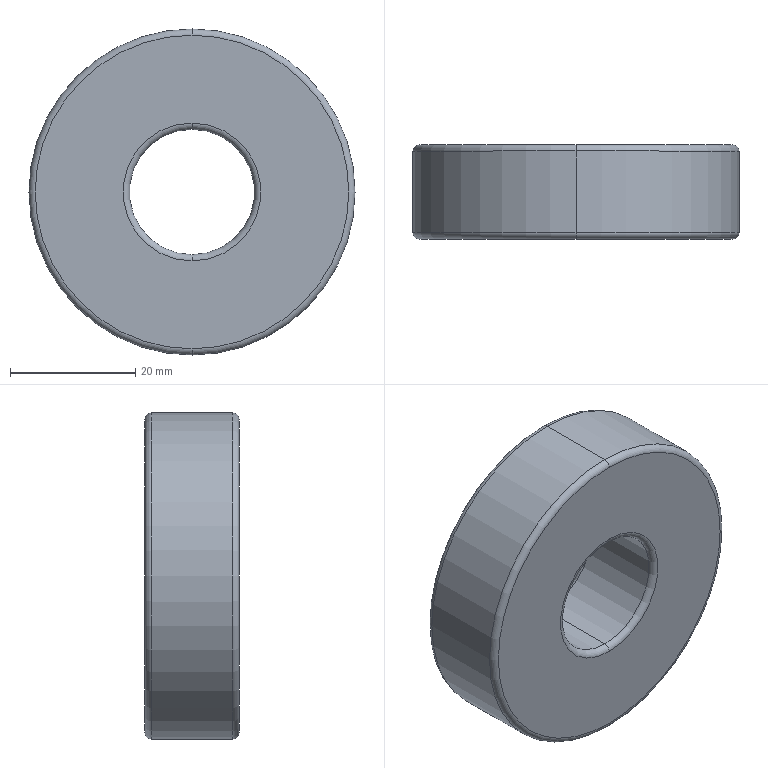Component | SolidWorks | BearingCH-NTN6304ZZ-1 | 1 solid | 14 faces | box 52 x 15 x 52 mm | volume 27046 mm3 | torus 8 | cylinder 4 | plane 2 | commonest cylinder face diameters 20 x2 52 x2
build123d program:
from build123d import *

# Parameters (mm, degrees)
SKETCH1_R           = 26
SKETCH1_R_2         = 10
BOSS_EXTRUDE1_DEPTH = 15
FILLET1_R           = 1


with BuildPart() as part:
    # Sketch1 → Boss-Extrude1 (new body)
    with BuildSketch(Plane(origin=(0, 0, 0), x_dir=(1, 0, 0), z_dir=(0, 1, 0))):
        with Locations(Location((0, 0, 0), (0, 0, 270))):
            Circle(SKETCH1_R)
        with Locations(Location((0, 0, 0), (0, 0, 270))):
            Circle(SKETCH1_R_2, mode=Mode.SUBTRACT)
    extrude(amount=BOSS_EXTRUDE1_DEPTH)

    # Fillet1
    fillet1_edges = [part.edges().sort_by_distance(p)[0] for p in [
        (0, 0, -26),
        (0, 15, -26),
        (0, 0, -10),
        (0, 15, -10),
    ]]
    fillet(fillet1_edges, radius=FILLET1_R)


solid = part.part

# Placed as in the assembly
solid = solid.moved(Location((-30.964, 101.813, 280.197), (0, 0, 0)))
STEP:
#1=COLOUR_RGB('',0.7922,0.8196,0.9333);
#2=FILL_AREA_STYLE_COLOUR('',#1);
#3=FILL_AREA_STYLE('',(#2));
#4=SURFACE_STYLE_FILL_AREA(#3);
#5=SURFACE_SIDE_STYLE('',(#4));
#6=SURFACE_STYLE_USAGE(.BOTH.,#5);
#7=PRESENTATION_STYLE_ASSIGNMENT((#6));
#8=CARTESIAN_POINT('',(-1.219,4.599,10.598));
#9=VERTEX_POINT('',#8);
#10=CARTESIAN_POINT('',(-1.219,4.599,11.464));
#11=VERTEX_POINT('',#10);
#12=CARTESIAN_POINT('',(-1.219,4.599,11.031));
#13=DIRECTION('',(0.,-1.,0.));
#14=DIRECTION('',(0.,0.,1.));
#15=AXIS2_PLACEMENT_3D('',#12,#13,#14);
#16=CIRCLE('',#15,0.4331);
#17=EDGE_CURVE('',#9,#11,#16,.T.);
#18=ORIENTED_EDGE('',*,*,#17,.F.);
#19=CARTESIAN_POINT('',(-1.219,4.56,10.638));
#20=VERTEX_POINT('',#19);
#21=CARTESIAN_POINT('',(-1.219,4.56,10.598));
#22=DIRECTION('',(1.,0.,0.));
#23=DIRECTION('',(0.,0.,-1.));
#24=AXIS2_PLACEMENT_3D('',#21,#22,#23);
#25=CIRCLE('',#24,0.03937);
#26=EDGE_CURVE('',#9,#20,#25,.T.);
#27=ORIENTED_EDGE('',*,*,#26,.T.);
#28=CARTESIAN_POINT('',(-1.219,4.56,11.425));
#29=VERTEX_POINT('',#28);
#30=CARTESIAN_POINT('',(-1.219,4.56,11.031));
#31=DIRECTION('',(0.,1.,0.));
#32=DIRECTION('',(0.,0.,1.));
#33=AXIS2_PLACEMENT_3D('',#30,#31,#32);
#34=CIRCLE('',#33,0.3937);
#35=EDGE_CURVE('',#29,#20,#34,.T.);
#36=ORIENTED_EDGE('',*,*,#35,.F.);
#37=CARTESIAN_POINT('',(-1.219,4.56,11.464));
#38=DIRECTION('',(-1.,0.,0.));
#39=DIRECTION('',(0.,0.,1.));
#40=AXIS2_PLACEMENT_3D('',#37,#38,#39);
#41=CIRCLE('',#40,0.03937);
#42=EDGE_CURVE('',#11,#29,#41,.T.);
#43=ORIENTED_EDGE('',*,*,#42,.F.);
#44=EDGE_LOOP('',(#18,#27,#36,#43));
#45=FACE_OUTER_BOUND('',#44,.T.);
#46=CARTESIAN_POINT('',(-1.219,4.56,11.031));
#47=DIRECTION('',(0.,1.,0.));
#48=DIRECTION('',(0.,0.,1.));
#49=AXIS2_PLACEMENT_3D('',#46,#47,#48);
#50=TOROIDAL_SURFACE('',#49,0.4331,0.03937);
#51=ADVANCED_FACE('',(#45),#50,.T.);
#52=CARTESIAN_POINT('',(-1.219,4.048,10.638));
#53=VERTEX_POINT('',#52);
#54=CARTESIAN_POINT('',(-1.219,4.048,11.425));
#55=VERTEX_POINT('',#54);
#56=CARTESIAN_POINT('',(-1.219,4.048,11.031));
#57=DIRECTION('',(0.,-1.,0.));
#58=DIRECTION('',(0.,0.,1.));
#59=AXIS2_PLACEMENT_3D('',#56,#57,#58);
#60=CIRCLE('',#59,0.3937);
#61=EDGE_CURVE('',#53,#55,#60,.T.);
#62=ORIENTED_EDGE('',*,*,#61,.F.);
#63=CARTESIAN_POINT('',(-1.219,4.008,10.598));
#64=VERTEX_POINT('',#63);
#65=CARTESIAN_POINT('',(-1.219,4.048,10.598));
#66=DIRECTION('',(1.,0.,0.));
#67=DIRECTION('',(0.,0.,-1.));
#68=AXIS2_PLACEMENT_3D('',#65,#66,#67);
#69=CIRCLE('',#68,0.03937);
#70=EDGE_CURVE('',#53,#64,#69,.T.);
#71=ORIENTED_EDGE('',*,*,#70,.T.);
#72=CARTESIAN_POINT('',(-1.219,4.008,11.464));
#73=VERTEX_POINT('',#72);
#74=CARTESIAN_POINT('',(-1.219,4.008,11.031));
#75=DIRECTION('',(0.,1.,0.));
#76=DIRECTION('',(0.,0.,1.));
#77=AXIS2_PLACEMENT_3D('',#74,#75,#76);
#78=CIRCLE('',#77,0.4331);
#79=EDGE_CURVE('',#73,#64,#78,.T.);
#80=ORIENTED_EDGE('',*,*,#79,.F.);
#81=CARTESIAN_POINT('',(-1.219,4.048,11.464));
#82=DIRECTION('',(-1.,0.,0.));
#83=DIRECTION('',(0.,0.,1.));
#84=AXIS2_PLACEMENT_3D('',#81,#82,#83);
#85=CIRCLE('',#84,0.03937);
#86=EDGE_CURVE('',#55,#73,#85,.T.);
#87=ORIENTED_EDGE('',*,*,#86,.F.);
#88=EDGE_LOOP('',(#62,#71,#80,#87));
#89=FACE_OUTER_BOUND('',#88,.T.);
#90=CARTESIAN_POINT('',(-1.219,4.048,11.031));
#91=DIRECTION('',(0.,1.,0.));
#92=DIRECTION('',(0.,0.,1.));
#93=AXIS2_PLACEMENT_3D('',#90,#91,#92);
#94=TOROIDAL_SURFACE('',#93,0.4331,0.03937);
#95=ADVANCED_FACE('',(#89),#94,.T.);
#96=CARTESIAN_POINT('',(-1.219,4.56,10.008));
#97=VERTEX_POINT('',#96);
#98=CARTESIAN_POINT('',(-1.219,4.56,12.055));
#99=VERTEX_POINT('',#98);
#100=CARTESIAN_POINT('',(-1.219,4.56,11.031));
#101=DIRECTION('',(0.,-1.,0.));
#102=DIRECTION('',(0.,0.,1.));
#103=AXIS2_PLACEMENT_3D('',#100,#101,#102);
#104=CIRCLE('',#103,1.024);
#105=EDGE_CURVE('',#97,#99,#104,.T.);
#106=ORIENTED_EDGE('',*,*,#105,.F.);
#107=CARTESIAN_POINT('',(-1.219,4.599,10.047));
#108=VERTEX_POINT('',#107);
#109=CARTESIAN_POINT('',(-1.219,4.56,10.047));
#110=DIRECTION('',(1.,0.,0.));
#111=DIRECTION('',(0.,0.,-1.));
#112=AXIS2_PLACEMENT_3D('',#109,#110,#111);
#113=CIRCLE('',#112,0.03937);
#114=EDGE_CURVE('',#97,#108,#113,.T.);
#115=ORIENTED_EDGE('',*,*,#114,.T.);
#116=CARTESIAN_POINT('',(-1.219,4.599,12.016));
#117=VERTEX_POINT('',#116);
#118=CARTESIAN_POINT('',(-1.219,4.599,11.031));
#119=DIRECTION('',(0.,1.,0.));
#120=DIRECTION('',(0.,0.,1.));
#121=AXIS2_PLACEMENT_3D('',#118,#119,#120);
#122=CIRCLE('',#121,0.9843);
#123=EDGE_CURVE('',#117,#108,#122,.T.);
#124=ORIENTED_EDGE('',*,*,#123,.F.);
#125=CARTESIAN_POINT('',(-1.219,4.56,12.016));
#126=DIRECTION('',(-1.,0.,0.));
#127=DIRECTION('',(0.,0.,1.));
#128=AXIS2_PLACEMENT_3D('',#125,#126,#127);
#129=CIRCLE('',#128,0.03937);
#130=EDGE_CURVE('',#99,#117,#129,.T.);
#131=ORIENTED_EDGE('',*,*,#130,.F.);
#132=EDGE_LOOP('',(#106,#115,#124,#131));
#133=FACE_OUTER_BOUND('',#132,.T.);
#134=CARTESIAN_POINT('',(-1.219,4.56,11.031));
#135=DIRECTION('',(0.,1.,0.));
#136=DIRECTION('',(0.,0.,1.));
#137=AXIS2_PLACEMENT_3D('',#134,#135,#136);
#138=TOROIDAL_SURFACE('',#137,0.9843,0.03937);
#139=ADVANCED_FACE('',(#133),#138,.T.);
#140=CARTESIAN_POINT('',(-1.219,4.008,10.047));
#141=VERTEX_POINT('',#140);
#142=CARTESIAN_POINT('',(-1.219,4.008,12.016));
#143=VERTEX_POINT('',#142);
#144=CARTESIAN_POINT('',(-1.219,4.008,11.031));
#145=DIRECTION('',(0.,-1.,0.));
#146=DIRECTION('',(0.,0.,1.));
#147=AXIS2_PLACEMENT_3D('',#144,#145,#146);
#148=CIRCLE('',#147,0.9843);
#149=EDGE_CURVE('',#141,#143,#148,.T.);
#150=ORIENTED_EDGE('',*,*,#149,.F.);
#151=CARTESIAN_POINT('',(-1.219,4.048,10.008));
#152=VERTEX_POINT('',#151);
#153=CARTESIAN_POINT('',(-1.219,4.048,10.047));
#154=DIRECTION('',(1.,0.,0.));
#155=DIRECTION('',(0.,0.,-1.));
#156=AXIS2_PLACEMENT_3D('',#153,#154,#155);
#157=CIRCLE('',#156,0.03937);
#158=EDGE_CURVE('',#141,#152,#157,.T.);
#159=ORIENTED_EDGE('',*,*,#158,.T.);
#160=CARTESIAN_POINT('',(-1.219,4.048,12.055));
#161=VERTEX_POINT('',#160);
#162=CARTESIAN_POINT('',(-1.219,4.048,11.031));
#163=DIRECTION('',(0.,1.,0.));
#164=DIRECTION('',(0.,0.,1.));
#165=AXIS2_PLACEMENT_3D('',#162,#163,#164);
#166=CIRCLE('',#165,1.024);
#167=EDGE_CURVE('',#161,#152,#166,.T.);
#168=ORIENTED_EDGE('',*,*,#167,.F.);
#169=CARTESIAN_POINT('',(-1.219,4.048,12.016));
#170=DIRECTION('',(-1.,0.,0.));
#171=DIRECTION('',(0.,0.,1.));
#172=AXIS2_PLACEMENT_3D('',#169,#170,#171);
#173=CIRCLE('',#172,0.03937);
#174=EDGE_CURVE('',#143,#161,#173,.T.);
#175=ORIENTED_EDGE('',*,*,#174,.F.);
#176=EDGE_LOOP('',(#150,#159,#168,#175));
#177=FACE_OUTER_BOUND('',#176,.T.);
#178=CARTESIAN_POINT('',(-1.219,4.048,11.031));
#179=DIRECTION('',(0.,1.,0.));
#180=DIRECTION('',(0.,0.,1.));
#181=AXIS2_PLACEMENT_3D('',#178,#179,#180);
#182=TOROIDAL_SURFACE('',#181,0.9843,0.03937);
#183=ADVANCED_FACE('',(#177),#182,.T.);
#184=CARTESIAN_POINT('',(-1.219,4.56,11.031));
#185=DIRECTION('',(0.,1.,0.));
#186=DIRECTION('',(0.,0.,1.));
#187=AXIS2_PLACEMENT_3D('',#184,#185,#186);
#188=CIRCLE('',#187,0.3937);
#189=EDGE_CURVE('',#20,#29,#188,.T.);
#190=ORIENTED_EDGE('',*,*,#189,.T.);
#191=CARTESIAN_POINT('',(-1.219,4.599,11.425));
#192=DIRECTION('',(0.,-1.,0.));
#193=VECTOR('',#192,39.37);
#194=LINE('',#191,#193);
#195=EDGE_CURVE('',#29,#55,#194,.T.);
#196=ORIENTED_EDGE('',*,*,#195,.T.);
#197=CARTESIAN_POINT('',(-1.219,4.048,11.031));
#198=DIRECTION('',(0.,-1.,0.));
#199=DIRECTION('',(0.,0.,1.));
#200=AXIS2_PLACEMENT_3D('',#197,#198,#199);
#201=CIRCLE('',#200,0.3937);
#202=EDGE_CURVE('',#55,#53,#201,.T.);
#203=ORIENTED_EDGE('',*,*,#202,.T.);
#204=CARTESIAN_POINT('',(-1.219,4.599,10.638));
#205=DIRECTION('',(0.,-1.,0.));
#206=VECTOR('',#205,39.37);
#207=LINE('',#204,#206);
#208=EDGE_CURVE('',#20,#53,#207,.T.);
#209=ORIENTED_EDGE('',*,*,#208,.F.);
#210=EDGE_LOOP('',(#190,#196,#203,#209));
#211=FACE_OUTER_BOUND('',#210,.T.);
#212=CARTESIAN_POINT('',(-1.219,4.599,11.031));
#213=DIRECTION('',(0.,-1.,0.));
#214=DIRECTION('',(0.,0.,-1.));
#215=AXIS2_PLACEMENT_3D('',#212,#213,#214);
#216=CYLINDRICAL_SURFACE('',#215,0.3937);
#217=ADVANCED_FACE('',(#211),#216,.F.);
#218=ORIENTED_EDGE('',*,*,#105,.T.);
#219=CARTESIAN_POINT('',(-1.219,4.599,12.055));
#220=DIRECTION('',(0.,-1.,0.));
#221=VECTOR('',#220,39.37);
#222=LINE('',#219,#221);
#223=EDGE_CURVE('',#99,#161,#222,.T.);
#224=ORIENTED_EDGE('',*,*,#223,.T.);
#225=ORIENTED_EDGE('',*,*,#167,.T.);
#226=CARTESIAN_POINT('',(-1.219,4.599,10.008));
#227=DIRECTION('',(0.,-1.,0.));
#228=VECTOR('',#227,39.37);
#229=LINE('',#226,#228);
#230=EDGE_CURVE('',#97,#152,#229,.T.);
#231=ORIENTED_EDGE('',*,*,#230,.F.);
#232=EDGE_LOOP('',(#218,#224,#225,#231));
#233=FACE_OUTER_BOUND('',#232,.T.);
#234=CARTESIAN_POINT('',(-1.219,4.599,11.031));
#235=DIRECTION('',(0.,-1.,0.));
#236=DIRECTION('',(0.,0.,-1.));
#237=AXIS2_PLACEMENT_3D('',#234,#235,#236);
#238=CYLINDRICAL_SURFACE('',#237,1.024);
#239=ADVANCED_FACE('',(#233),#238,.T.);
#240=ORIENTED_EDGE('',*,*,#123,.T.);
#241=CARTESIAN_POINT('',(-1.219,4.599,11.031));
#242=DIRECTION('',(0.,1.,0.));
#243=DIRECTION('',(0.,0.,1.));
#244=AXIS2_PLACEMENT_3D('',#241,#242,#243);
#245=CIRCLE('',#244,0.9843);
#246=EDGE_CURVE('',#108,#117,#245,.T.);
#247=ORIENTED_EDGE('',*,*,#246,.T.);
#248=EDGE_LOOP('',(#240,#247));
#249=FACE_OUTER_BOUND('',#248,.T.);
#250=CARTESIAN_POINT('',(-1.219,4.599,11.031));
#251=DIRECTION('',(0.,-1.,0.));
#252=DIRECTION('',(0.,0.,1.));
#253=AXIS2_PLACEMENT_3D('',#250,#251,#252);
#254=CIRCLE('',#253,0.4331);
#255=EDGE_CURVE('',#11,#9,#254,.T.);
#256=ORIENTED_EDGE('',*,*,#255,.T.);
#257=ORIENTED_EDGE('',*,*,#17,.T.);
#258=EDGE_LOOP('',(#256,#257));
#259=FACE_BOUND('',#258,.T.);
#260=CARTESIAN_POINT('',(-1.219,4.599,11.031));
#261=DIRECTION('',(0.,1.,0.));
#262=DIRECTION('',(0.,0.,1.));
#263=AXIS2_PLACEMENT_3D('',#260,#261,#262);
#264=PLANE('',#263);
#265=ADVANCED_FACE('',(#249,#259),#264,.T.);
#266=CARTESIAN_POINT('',(-1.219,4.008,11.031));
#267=DIRECTION('',(0.,-1.,0.));
#268=DIRECTION('',(0.,0.,1.));
#269=AXIS2_PLACEMENT_3D('',#266,#267,#268);
#270=CIRCLE('',#269,0.9843);
#271=EDGE_CURVE('',#143,#141,#270,.T.);
#272=ORIENTED_EDGE('',*,*,#271,.T.);
#273=ORIENTED_EDGE('',*,*,#149,.T.);
#274=EDGE_LOOP('',(#272,#273));
#275=FACE_OUTER_BOUND('',#274,.T.);
#276=ORIENTED_EDGE('',*,*,#79,.T.);
#277=CARTESIAN_POINT('',(-1.219,4.008,11.031));
#278=DIRECTION('',(0.,1.,0.));
#279=DIRECTION('',(0.,0.,1.));
#280=AXIS2_PLACEMENT_3D('',#277,#278,#279);
#281=CIRCLE('',#280,0.4331);
#282=EDGE_CURVE('',#64,#73,#281,.T.);
#283=ORIENTED_EDGE('',*,*,#282,.T.);
#284=EDGE_LOOP('',(#276,#283));
#285=FACE_BOUND('',#284,.T.);
#286=CARTESIAN_POINT('',(-1.219,4.008,11.031));
#287=DIRECTION('',(0.,1.,0.));
#288=DIRECTION('',(0.,0.,1.));
#289=AXIS2_PLACEMENT_3D('',#286,#287,#288);
#290=PLANE('',#289);
#291=ADVANCED_FACE('',(#275,#285),#290,.F.);
#292=ORIENTED_EDGE('',*,*,#223,.F.);
#293=CARTESIAN_POINT('',(-1.219,4.56,11.031));
#294=DIRECTION('',(0.,-1.,0.));
#295=DIRECTION('',(0.,0.,1.));
#296=AXIS2_PLACEMENT_3D('',#293,#294,#295);
#297=CIRCLE('',#296,1.024);
#298=EDGE_CURVE('',#99,#97,#297,.T.);
#299=ORIENTED_EDGE('',*,*,#298,.T.);
#300=ORIENTED_EDGE('',*,*,#230,.T.);
#301=CARTESIAN_POINT('',(-1.219,4.048,11.031));
#302=DIRECTION('',(0.,1.,0.));
#303=DIRECTION('',(0.,0.,1.));
#304=AXIS2_PLACEMENT_3D('',#301,#302,#303);
#305=CIRCLE('',#304,1.024);
#306=EDGE_CURVE('',#152,#161,#305,.T.);
#307=ORIENTED_EDGE('',*,*,#306,.T.);
#308=EDGE_LOOP('',(#292,#299,#300,#307));
#309=FACE_OUTER_BOUND('',#308,.T.);
#310=CARTESIAN_POINT('',(-1.219,4.599,11.031));
#311=DIRECTION('',(0.,-1.,0.));
#312=DIRECTION('',(0.,0.,-1.));
#313=AXIS2_PLACEMENT_3D('',#310,#311,#312);
#314=CYLINDRICAL_SURFACE('',#313,1.024);
#315=ADVANCED_FACE('',(#309),#314,.T.);
#316=ORIENTED_EDGE('',*,*,#195,.F.);
#317=ORIENTED_EDGE('',*,*,#35,.T.);
#318=ORIENTED_EDGE('',*,*,#208,.T.);
#319=ORIENTED_EDGE('',*,*,#61,.T.);
#320=EDGE_LOOP('',(#316,#317,#318,#319));
#321=FACE_OUTER_BOUND('',#320,.T.);
#322=CARTESIAN_POINT('',(-1.219,4.599,11.031));
#323=DIRECTION('',(0.,-1.,0.));
#324=DIRECTION('',(0.,0.,-1.));
#325=AXIS2_PLACEMENT_3D('',#322,#323,#324);
#326=CYLINDRICAL_SURFACE('',#325,0.3937);
#327=ADVANCED_FACE('',(#321),#326,.F.);
#328=ORIENTED_EDGE('',*,*,#158,.F.);
#329=ORIENTED_EDGE('',*,*,#271,.F.);
#330=ORIENTED_EDGE('',*,*,#174,.T.);
#331=ORIENTED_EDGE('',*,*,#306,.F.);
#332=EDGE_LOOP('',(#328,#329,#330,#331));
#333=FACE_OUTER_BOUND('',#332,.T.);
#334=CARTESIAN_POINT('',(-1.219,4.048,11.031));
#335=DIRECTION('',(0.,1.,0.));
#336=DIRECTION('',(0.,0.,1.));
#337=AXIS2_PLACEMENT_3D('',#334,#335,#336);
#338=TOROIDAL_SURFACE('',#337,0.9843,0.03937);
#339=ADVANCED_FACE('',(#333),#338,.T.);
#340=ORIENTED_EDGE('',*,*,#114,.F.);
#341=ORIENTED_EDGE('',*,*,#298,.F.);
#342=ORIENTED_EDGE('',*,*,#130,.T.);
#343=ORIENTED_EDGE('',*,*,#246,.F.);
#344=EDGE_LOOP('',(#340,#341,#342,#343));
#345=FACE_OUTER_BOUND('',#344,.T.);
#346=CARTESIAN_POINT('',(-1.219,4.56,11.031));
#347=DIRECTION('',(0.,1.,0.));
#348=DIRECTION('',(0.,0.,1.));
#349=AXIS2_PLACEMENT_3D('',#346,#347,#348);
#350=TOROIDAL_SURFACE('',#349,0.9843,0.03937);
#351=ADVANCED_FACE('',(#345),#350,.T.);
#352=ORIENTED_EDGE('',*,*,#70,.F.);
#353=ORIENTED_EDGE('',*,*,#202,.F.);
#354=ORIENTED_EDGE('',*,*,#86,.T.);
#355=ORIENTED_EDGE('',*,*,#282,.F.);
#356=EDGE_LOOP('',(#352,#353,#354,#355));
#357=FACE_OUTER_BOUND('',#356,.T.);
#358=CARTESIAN_POINT('',(-1.219,4.048,11.031));
#359=DIRECTION('',(0.,1.,0.));
#360=DIRECTION('',(0.,0.,1.));
#361=AXIS2_PLACEMENT_3D('',#358,#359,#360);
#362=TOROIDAL_SURFACE('',#361,0.4331,0.03937);
#363=ADVANCED_FACE('',(#357),#362,.T.);
#364=ORIENTED_EDGE('',*,*,#26,.F.);
#365=ORIENTED_EDGE('',*,*,#255,.F.);
#366=ORIENTED_EDGE('',*,*,#42,.T.);
#367=ORIENTED_EDGE('',*,*,#189,.F.);
#368=EDGE_LOOP('',(#364,#365,#366,#367));
#369=FACE_OUTER_BOUND('',#368,.T.);
#370=CARTESIAN_POINT('',(-1.219,4.56,11.031));
#371=DIRECTION('',(0.,1.,0.));
#372=DIRECTION('',(0.,0.,1.));
#373=AXIS2_PLACEMENT_3D('',#370,#371,#372);
#374=TOROIDAL_SURFACE('',#373,0.4331,0.03937);
#375=ADVANCED_FACE('',(#369),#374,.T.);
#376=CLOSED_SHELL('',(#51,#95,#139,#183,#217,#239,#265,#291,#315,#327,#339,#351,#363,#375));
#377=MANIFOLD_SOLID_BREP('',#376);
#378=STYLED_ITEM('',(#7),#377);
#379=PRESENTATION_LAYER_ASSIGNMENT('','',(#378));
#380=CARTESIAN_POINT('',(0.,0.,0.));
#381=DIRECTION('',(0.,0.,1.));
#382=DIRECTION('',(1.,0.,0.));
#383=AXIS2_PLACEMENT_3D('',#380,#381,#382);
#384=(LENGTH_UNIT()NAMED_UNIT(*)SI_UNIT($,.METRE.));
#385=LENGTH_MEASURE_WITH_UNIT(LENGTH_MEASURE(0.0254),#384);
#386=DIMENSIONAL_EXPONENTS(1.,0.,0.,0.,0.,0.,0.);
#387=(CONVERSION_BASED_UNIT('',#385)LENGTH_UNIT()NAMED_UNIT(#386));
#388=UNCERTAINTY_MEASURE_WITH_UNIT(LENGTH_MEASURE(0.00001),#387,'','');
#389=(NAMED_UNIT(*)PLANE_ANGLE_UNIT()SI_UNIT($,.RADIAN.));
#390=(NAMED_UNIT(*)SI_UNIT($,.STERADIAN.)SOLID_ANGLE_UNIT());
#391=(GEOMETRIC_REPRESENTATION_CONTEXT(3)GLOBAL_UNCERTAINTY_ASSIGNED_CONTEXT((#388))GLOBAL_UNIT_ASSIGNED_CONTEXT((#387,#389,#390))REPRESENTATION_CONTEXT('',''));
#392=ADVANCED_BREP_SHAPE_REPRESENTATION('',(#377,#383),#391);
#393=(LENGTH_UNIT()NAMED_UNIT(*)SI_UNIT($,.METRE.));
#394=LENGTH_MEASURE_WITH_UNIT(LENGTH_MEASURE(0.0254),#393);
#395=DIMENSIONAL_EXPONENTS(1.,0.,0.,0.,0.,0.,0.);
#396=(CONVERSION_BASED_UNIT('',#394)LENGTH_UNIT()NAMED_UNIT(#395));
#397=UNCERTAINTY_MEASURE_WITH_UNIT(LENGTH_MEASURE(0.00001),#396,'','');
#398=(NAMED_UNIT(*)PLANE_ANGLE_UNIT()SI_UNIT($,.RADIAN.));
#399=(NAMED_UNIT(*)SI_UNIT($,.STERADIAN.)SOLID_ANGLE_UNIT());
#400=(GEOMETRIC_REPRESENTATION_CONTEXT(3)GLOBAL_UNCERTAINTY_ASSIGNED_CONTEXT((#397))GLOBAL_UNIT_ASSIGNED_CONTEXT((#396,#398,#399))REPRESENTATION_CONTEXT('',''));
#401=MECHANICAL_DESIGN_GEOMETRIC_PRESENTATION_REPRESENTATION('',(#378),#400);